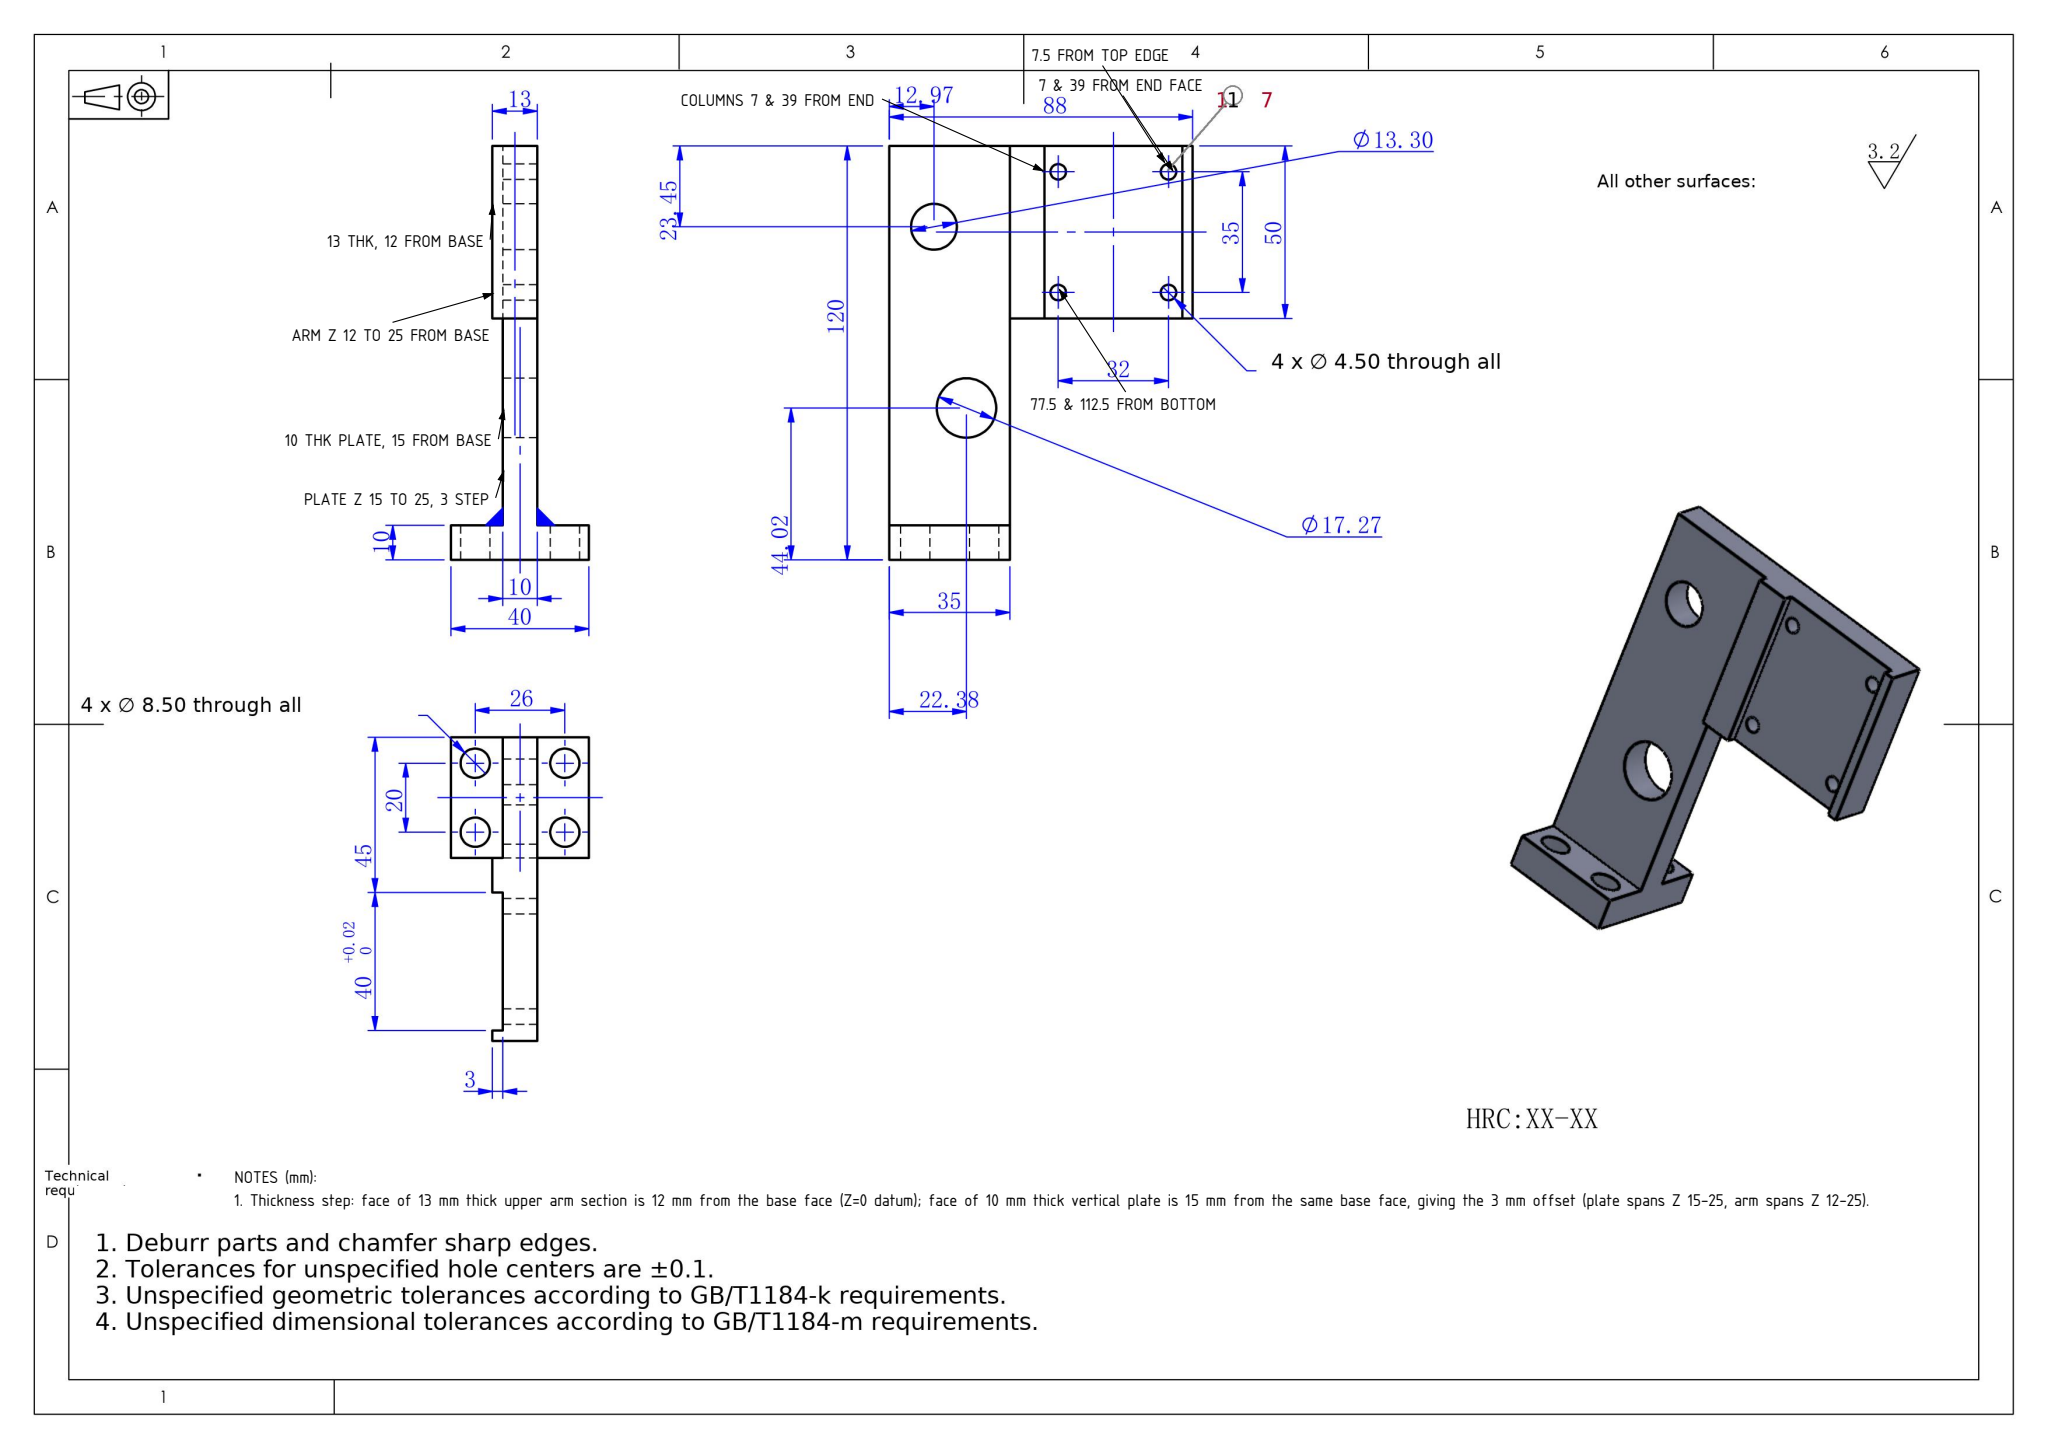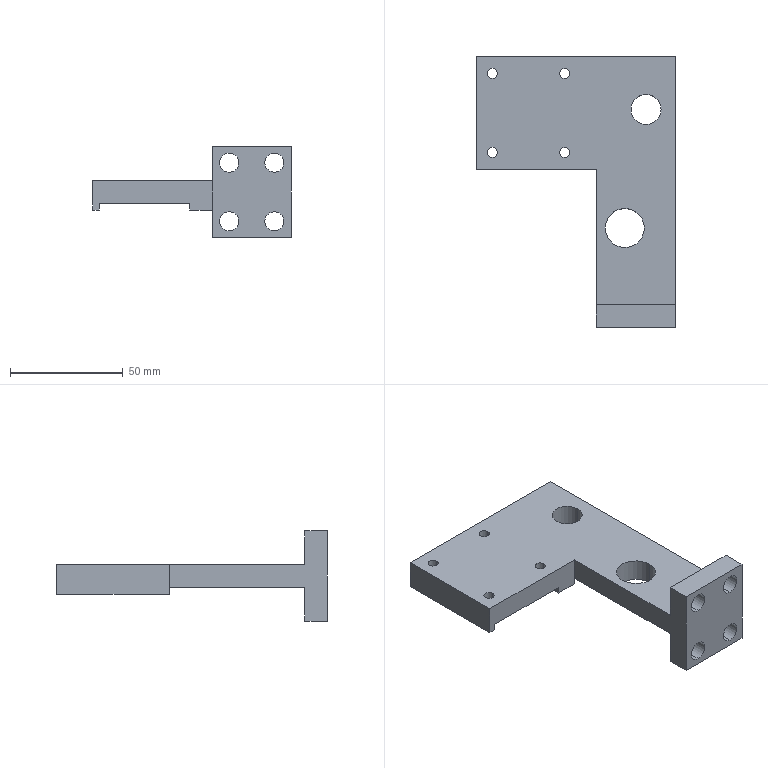Part | SolidWorks | mm | 1 solid | 38 faces | box 88 x 120 x 40 mm | volume 74314 mm3 | cylinder 20 | plane 18 | commonest cylinder face diameters 8.5 x8 4.5 x8 13.297 x2 17.267 x2
Drawing notes:
4X Ø4.50 THRU ALL: hole pattern located 7 mm from the left end face (X=0 datum) to first column, 32 mm to second column (X=7 and X=39); rows at 77.5 and 112.5 from the bottom face (Y=0 datum), 35 mm apart. | from the solid: cylinders dia 4.5 axis z at (7,77.5), (7,112.5), (39,77.5), (39,112.5), length 10; planes x=0, y=0
Thickness step: face of 13 mm thick upper arm section is 12 mm from the base face (Z=0 datum); face of 10 mm thick vertical plate is 15 mm from the same base face, giving the 3 mm offset (plate spans Z 15-25, arm spans Z 12-25). | from the solid: axis_planes z = 0.0, 12.0, 15.0, 25.0, 40.0
4X Ø4.50 THRU ALL: hole pattern 32 mm (along arm length) x 35 mm; nearest hole centers located 7 mm from the end face of the arm (datum: x=0 face) and 7.5 mm from the outer face at y=120. | from the solid: cylinders dia 4.5 axis z at (x,y) = (7,77.5), (39,77.5), (7,112.5), (39,112.5); bbox_xyz 88 x 120 x 40
13 mm thick upper arm section is located 12 mm from the base face (plane z=0) and ends at z=25; i.e. offset 12 mm from the 40 mm wide base face. | from the solid: axis_planes z = 0.0, 12.0, 25.0, 40.0
10 mm thick vertical plate is located 15 mm from the base face (plane z=0) and ends at z=25, giving the 3 mm step relative to the 13 mm arm section. | from the solid: axis_planes z = 0.0, 15.0, 25.0
4X Ø4.50 THRU ALL: hole column centers located 7 mm and 39 mm from the x=0 end face (32 mm apart); rows at 77.5 mm and 112.5 mm from the y=0 bottom face (35 mm apart). | from the solid: cylinders dia 4.5 axis z at (7.0,77.5), (7.0,112.5), (39.0,77.5), (39.0,112.5)
13 mm thick upper arm section spans z=12 to z=25 from the base face z=0 (40 mm overall width). | from the solid: axis_planes z=12.0 and z=25.0; bbox_xyz z=40
10 mm thick vertical plate spans z=15 to z=25 from the base face z=0, giving a 3 mm step from the 13 mm arm section. | from the solid: axis_planes z=15.0 and z=25.0
4X Ø4.50 THRU ALL: hole columns 7 and 39 from the x=0 end face of the arm; rows 77.5 and 112.5 from the y=0 bottom face (32 x 35 pattern). | from the solid: cylinders hole/bore d4.5 axis z at (7.0,77.5), (7.0,112.5), (39.0,77.5), (39.0,112.5), from z=15 to z=25
build123d program:
from build123d import *

# Parameters (mm, degrees)
BOSS_EXTRUDE1_DEPTH        = 10
SKETCH2_W                  = 35
SKETCH2_H                  = 40
BOSS_EXTRUDE2_DEPTH        = 10
SKETCH3_W                  = 13
SKETCH3_H                  = 50
BOSS_EXTRUDE3_DEPTH        = 3
SKETCH4_W                  = 10
SKETCH4_H                  = 50
BOSS_EXTRUDE4_DEPTH        = 3
F_4_5_4_5_DIAMETER_HOLE1_D = 4.5
F_8_5_8_5_DIAMETER_HOLE1_D = 8.5
SKETCH12_R                 = 6.649
SKETCH12_R_2               = 8.633
CUT_EXTRUDE1_DEPTH         = 34


with BuildPart() as part:
    # Sketch1 → Boss-Extrude1 (new body)
    with BuildSketch(Plane.XY):
        Polygon((-81.089, 4.223), (-31.089, 4.223), (-31.089, -55.777), (3.911, -55.777), (3.911, 54.223), (-81.089, 54.223), align=None)
    extrude(amount=BOSS_EXTRUDE1_DEPTH)

    # Sketch2 → Boss-Extrude2 (add)
    with BuildSketch(Plane(origin=(0, -55.777, 0), x_dir=(-1, 0, 0), z_dir=(0, -1, 0))):
        with Locations((13.589, -5)):
            Rectangle(SKETCH2_W, SKETCH2_H)
    extrude(amount=BOSS_EXTRUDE2_DEPTH)

    # Sketch3 → Boss-Extrude3 (add)
    with BuildSketch(Plane.ZY.offset(81.089)):
        with Locations((3.5, 29.223)):
            Rectangle(SKETCH3_W, SKETCH3_H)
    extrude(amount=BOSS_EXTRUDE3_DEPTH)

    # Sketch4 → Boss-Extrude4 (add)
    with BuildSketch(Plane(origin=(0, 0, 0), x_dir=(-1, 0, 0), z_dir=(0, 0, -1))):
        with Locations((36.089, 29.223)):
            Rectangle(SKETCH4_W, SKETCH4_H)
    extrude(amount=BOSS_EXTRUDE4_DEPTH)

    # 4.5 _4.5_ Diameter Hole1 (through all)
    with Locations(Plane.XY.offset(10)):
        with Locations((-77.089, 46.723), (-45.089, 46.723), (-77.089, 11.723), (-45.089, 11.723)):
            Hole(F_4_5_4_5_DIAMETER_HOLE1_D / 2)

    # 8.5 _8.5_ Diameter Hole1 (through all)
    with Locations(Plane(origin=(0, -55.777, 0), x_dir=(1, 0, 0), z_dir=(0, 1, 0))):
        with Locations((-23.589, 8), (-3.589, 8), (-23.589, -18), (-3.589, -18)):
            Hole(F_8_5_8_5_DIAMETER_HOLE1_D / 2)

    # Sketch12 → Cut-Extrude1 (cut)
    with BuildSketch(Plane(origin=(0, 0, 0), x_dir=(-1, 0, 0), z_dir=(0, 0, -1))):
        with Locations((9.055, 30.778)):
            Circle(SKETCH12_R)
        with Locations((18.47, -21.758)):
            Circle(SKETCH12_R_2)
    extrude(amount=-CUT_EXTRUDE1_DEPTH, mode=Mode.SUBTRACT)


solid = part.part